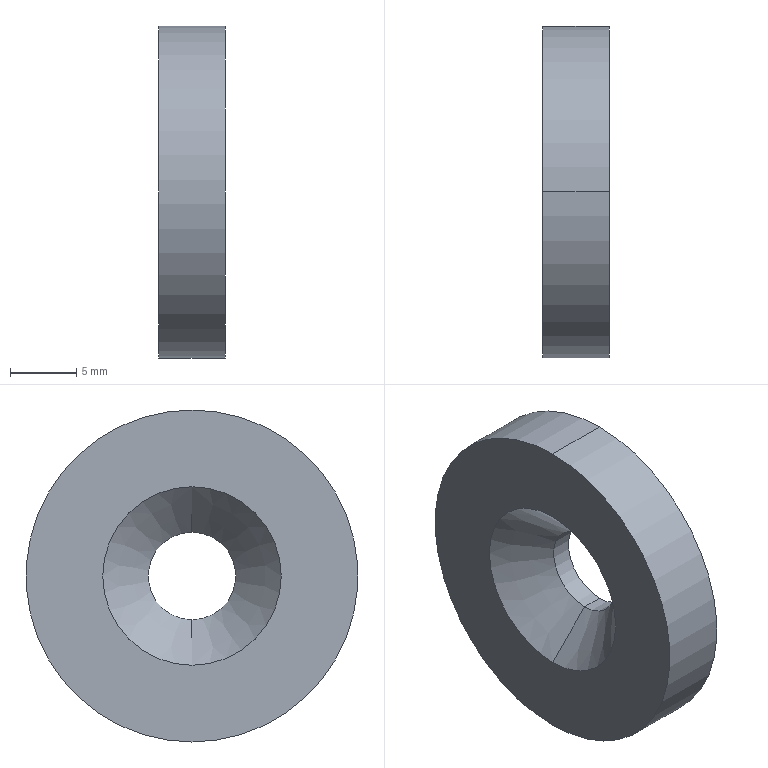Component | SolidWorks | EndCap1-1 | 1 solid | 8 faces | box 5 x 25 x 25 mm | volume 2120 mm3 | cylinder 4 | cone 2 | plane 2 | commonest cylinder face diameters 6.6 x2 25 x2
build123d program:
from build123d import *

# Parameters (mm, degrees)
SKETCH1_R                                            = 12.5
BOSS_EXTRUDE1_DEPTH                                  = 5
COUNTERSUNK_HOLE_FOR_M6_HEXAGON_SOCKET_C_D           = 6.6
COUNTERSUNK_HOLE_FOR_M6_HEXAGON_SOCKET_C_DEPTH       = 15
COUNTERSUNK_HOLE_FOR_M6_HEXAGON_SOCKET_C_CSINK_D     = 13.44
COUNTERSUNK_HOLE_FOR_M6_HEXAGON_SOCKET_C_CSINK_ANGLE = 90
COUNTERSUNK_HOLE_FOR_M6_HEXAGON_SOCKET_C_TIP         = 1.983


with BuildPart() as part:
    # Sketch1 → Boss-Extrude1 (new body)
    with BuildSketch(Plane.XY):
        Circle(SKETCH1_R)
    extrude(amount=BOSS_EXTRUDE1_DEPTH)

    # Countersunk Hole for M6 Hexagon Socket C
    with Locations(Plane.XY.offset(5)):
        with Locations((0, 0)):
            CounterSinkHole(COUNTERSUNK_HOLE_FOR_M6_HEXAGON_SOCKET_C_D / 2, COUNTERSUNK_HOLE_FOR_M6_HEXAGON_SOCKET_C_CSINK_D / 2, depth=COUNTERSUNK_HOLE_FOR_M6_HEXAGON_SOCKET_C_DEPTH, counter_sink_angle=COUNTERSUNK_HOLE_FOR_M6_HEXAGON_SOCKET_C_CSINK_ANGLE)
            with Locations((0, 0, -(COUNTERSUNK_HOLE_FOR_M6_HEXAGON_SOCKET_C_DEPTH + COUNTERSUNK_HOLE_FOR_M6_HEXAGON_SOCKET_C_TIP / 2))):  # 118° drill point
                Cone(0, COUNTERSUNK_HOLE_FOR_M6_HEXAGON_SOCKET_C_D / 2, COUNTERSUNK_HOLE_FOR_M6_HEXAGON_SOCKET_C_TIP, mode=Mode.SUBTRACT)


solid = part.part

# Placed as in the assembly
solid = solid.moved(Location((181.468, -65.334, 2056.399), (0, -90, 0)))
STEP:
#1=CARTESIAN_POINT('',(7.082,-2.572,80.831));
#2=VERTEX_POINT('',#1);
#3=CARTESIAN_POINT('',(7.082,-2.572,81.091));
#4=VERTEX_POINT('',#3);
#5=CARTESIAN_POINT('',(7.082,-2.572,80.961));
#6=DIRECTION('',(-1.,0.,-0.));
#7=DIRECTION('',(0.,0.,1.));
#8=AXIS2_PLACEMENT_3D('',#5,#6,#7);
#9=CIRCLE('',#8,0.1299);
#10=EDGE_CURVE('',#2,#4,#9,.T.);
#11=ORIENTED_EDGE('',*,*,#10,.F.);
#12=CARTESIAN_POINT('',(6.948,-2.572,80.696));
#13=VERTEX_POINT('',#12);
#14=CARTESIAN_POINT('',(6.948,-2.572,80.696));
#15=DIRECTION('',(-0.7071,0.,-0.7071));
#16=VECTOR('',#15,39.37);
#17=LINE('',#14,#16);
#18=EDGE_CURVE('',#2,#13,#17,.T.);
#19=ORIENTED_EDGE('',*,*,#18,.T.);
#20=CARTESIAN_POINT('',(6.948,-2.572,81.225));
#21=VERTEX_POINT('',#20);
#22=CARTESIAN_POINT('',(6.948,-2.572,80.961));
#23=DIRECTION('',(-1.,0.,-0.));
#24=DIRECTION('',(0.,0.,1.));
#25=AXIS2_PLACEMENT_3D('',#22,#23,#24);
#26=CIRCLE('',#25,0.2646);
#27=EDGE_CURVE('',#13,#21,#26,.T.);
#28=ORIENTED_EDGE('',*,*,#27,.T.);
#29=CARTESIAN_POINT('',(6.948,-2.572,81.225));
#30=DIRECTION('',(-0.7071,0.,0.7071));
#31=VECTOR('',#30,39.37);
#32=LINE('',#29,#31);
#33=EDGE_CURVE('',#4,#21,#32,.T.);
#34=ORIENTED_EDGE('',*,*,#33,.F.);
#35=EDGE_LOOP('',(#11,#19,#28,#34));
#36=FACE_OUTER_BOUND('',#35,.T.);
#37=CARTESIAN_POINT('',(6.948,-2.572,80.961));
#38=DIRECTION('',(-1.,0.,-0.));
#39=DIRECTION('',(0.,0.,1.));
#40=AXIS2_PLACEMENT_3D('',#37,#38,#39);
#41=CONICAL_SURFACE('',#40,0.2646,0.7854);
#42=ADVANCED_FACE('',(#36),#41,.F.);
#43=CARTESIAN_POINT('',(7.144,-2.572,80.831));
#44=VERTEX_POINT('',#43);
#45=CARTESIAN_POINT('',(7.144,-2.572,81.091));
#46=VERTEX_POINT('',#45);
#47=CARTESIAN_POINT('',(7.144,-2.572,80.961));
#48=DIRECTION('',(-1.,0.,-0.));
#49=DIRECTION('',(0.,0.,1.));
#50=AXIS2_PLACEMENT_3D('',#47,#48,#49);
#51=CIRCLE('',#50,0.1299);
#52=EDGE_CURVE('',#44,#46,#51,.T.);
#53=ORIENTED_EDGE('',*,*,#52,.F.);
#54=CARTESIAN_POINT('',(6.948,-2.572,80.831));
#55=DIRECTION('',(-1.,0.,-0.));
#56=VECTOR('',#55,39.37);
#57=LINE('',#54,#56);
#58=EDGE_CURVE('',#44,#2,#57,.T.);
#59=ORIENTED_EDGE('',*,*,#58,.T.);
#60=ORIENTED_EDGE('',*,*,#10,.T.);
#61=CARTESIAN_POINT('',(6.948,-2.572,81.091));
#62=DIRECTION('',(-1.,0.,-0.));
#63=VECTOR('',#62,39.37);
#64=LINE('',#61,#63);
#65=EDGE_CURVE('',#46,#4,#64,.T.);
#66=ORIENTED_EDGE('',*,*,#65,.F.);
#67=EDGE_LOOP('',(#53,#59,#60,#66));
#68=FACE_OUTER_BOUND('',#67,.T.);
#69=CARTESIAN_POINT('',(6.948,-2.572,80.961));
#70=DIRECTION('',(-1.,0.,-0.));
#71=DIRECTION('',(0.,0.,1.));
#72=AXIS2_PLACEMENT_3D('',#69,#70,#71);
#73=CYLINDRICAL_SURFACE('',#72,0.1299);
#74=ADVANCED_FACE('',(#68),#73,.F.);
#75=CARTESIAN_POINT('',(6.948,-2.572,81.453));
#76=VERTEX_POINT('',#75);
#77=CARTESIAN_POINT('',(6.948,-2.572,80.468));
#78=VERTEX_POINT('',#77);
#79=CARTESIAN_POINT('',(6.948,-2.572,80.961));
#80=DIRECTION('',(-1.,0.,-0.));
#81=DIRECTION('',(0.,0.,1.));
#82=AXIS2_PLACEMENT_3D('',#79,#80,#81);
#83=CIRCLE('',#82,0.4921);
#84=EDGE_CURVE('',#76,#78,#83,.T.);
#85=ORIENTED_EDGE('',*,*,#84,.F.);
#86=CARTESIAN_POINT('',(7.144,-2.572,81.453));
#87=VERTEX_POINT('',#86);
#88=CARTESIAN_POINT('',(6.948,-2.572,81.453));
#89=DIRECTION('',(1.,-0.,0.));
#90=VECTOR('',#89,39.37);
#91=LINE('',#88,#90);
#92=EDGE_CURVE('',#76,#87,#91,.T.);
#93=ORIENTED_EDGE('',*,*,#92,.T.);
#94=CARTESIAN_POINT('',(7.144,-2.572,80.468));
#95=VERTEX_POINT('',#94);
#96=CARTESIAN_POINT('',(7.144,-2.572,80.961));
#97=DIRECTION('',(-1.,0.,-0.));
#98=DIRECTION('',(0.,0.,1.));
#99=AXIS2_PLACEMENT_3D('',#96,#97,#98);
#100=CIRCLE('',#99,0.4921);
#101=EDGE_CURVE('',#87,#95,#100,.T.);
#102=ORIENTED_EDGE('',*,*,#101,.T.);
#103=CARTESIAN_POINT('',(6.948,-2.572,80.468));
#104=DIRECTION('',(1.,-0.,0.));
#105=VECTOR('',#104,39.37);
#106=LINE('',#103,#105);
#107=EDGE_CURVE('',#78,#95,#106,.T.);
#108=ORIENTED_EDGE('',*,*,#107,.F.);
#109=EDGE_LOOP('',(#85,#93,#102,#108));
#110=FACE_OUTER_BOUND('',#109,.T.);
#111=CARTESIAN_POINT('',(6.948,-2.572,80.961));
#112=DIRECTION('',(1.,-0.,0.));
#113=DIRECTION('',(0.,0.,-1.));
#114=AXIS2_PLACEMENT_3D('',#111,#112,#113);
#115=CYLINDRICAL_SURFACE('',#114,0.4921);
#116=ADVANCED_FACE('',(#110),#115,.T.);
#117=ORIENTED_EDGE('',*,*,#92,.F.);
#118=CARTESIAN_POINT('',(6.948,-2.572,80.961));
#119=DIRECTION('',(-1.,0.,-0.));
#120=DIRECTION('',(0.,0.,1.));
#121=AXIS2_PLACEMENT_3D('',#118,#119,#120);
#122=CIRCLE('',#121,0.4921);
#123=EDGE_CURVE('',#78,#76,#122,.T.);
#124=ORIENTED_EDGE('',*,*,#123,.F.);
#125=ORIENTED_EDGE('',*,*,#107,.T.);
#126=CARTESIAN_POINT('',(7.144,-2.572,80.961));
#127=DIRECTION('',(-1.,0.,-0.));
#128=DIRECTION('',(0.,0.,1.));
#129=AXIS2_PLACEMENT_3D('',#126,#127,#128);
#130=CIRCLE('',#129,0.4921);
#131=EDGE_CURVE('',#95,#87,#130,.T.);
#132=ORIENTED_EDGE('',*,*,#131,.T.);
#133=EDGE_LOOP('',(#117,#124,#125,#132));
#134=FACE_OUTER_BOUND('',#133,.T.);
#135=CARTESIAN_POINT('',(6.948,-2.572,80.961));
#136=DIRECTION('',(1.,-0.,0.));
#137=DIRECTION('',(0.,0.,-1.));
#138=AXIS2_PLACEMENT_3D('',#135,#136,#137);
#139=CYLINDRICAL_SURFACE('',#138,0.4921);
#140=ADVANCED_FACE('',(#134),#139,.T.);
#141=CARTESIAN_POINT('',(6.948,-2.572,80.961));
#142=DIRECTION('',(-1.,0.,-0.));
#143=DIRECTION('',(0.,0.,1.));
#144=AXIS2_PLACEMENT_3D('',#141,#142,#143);
#145=CIRCLE('',#144,0.2646);
#146=EDGE_CURVE('',#21,#13,#145,.T.);
#147=ORIENTED_EDGE('',*,*,#146,.F.);
#148=ORIENTED_EDGE('',*,*,#27,.F.);
#149=EDGE_LOOP('',(#147,#148));
#150=FACE_BOUND('',#149,.T.);
#151=ORIENTED_EDGE('',*,*,#123,.T.);
#152=ORIENTED_EDGE('',*,*,#84,.T.);
#153=EDGE_LOOP('',(#151,#152));
#154=FACE_OUTER_BOUND('',#153,.T.);
#155=CARTESIAN_POINT('',(6.948,-2.572,80.961));
#156=DIRECTION('',(-1.,0.,-0.));
#157=DIRECTION('',(-0.,0.,1.));
#158=AXIS2_PLACEMENT_3D('',#155,#156,#157);
#159=PLANE('',#158);
#160=ADVANCED_FACE('',(#150,#154),#159,.T.);
#161=CARTESIAN_POINT('',(7.144,-2.572,80.961));
#162=DIRECTION('',(-1.,0.,-0.));
#163=DIRECTION('',(0.,0.,1.));
#164=AXIS2_PLACEMENT_3D('',#161,#162,#163);
#165=CIRCLE('',#164,0.1299);
#166=EDGE_CURVE('',#46,#44,#165,.T.);
#167=ORIENTED_EDGE('',*,*,#166,.T.);
#168=ORIENTED_EDGE('',*,*,#52,.T.);
#169=EDGE_LOOP('',(#167,#168));
#170=FACE_BOUND('',#169,.T.);
#171=ORIENTED_EDGE('',*,*,#131,.F.);
#172=ORIENTED_EDGE('',*,*,#101,.F.);
#173=EDGE_LOOP('',(#171,#172));
#174=FACE_OUTER_BOUND('',#173,.T.);
#175=CARTESIAN_POINT('',(7.144,-2.572,80.961));
#176=DIRECTION('',(-1.,0.,-0.));
#177=DIRECTION('',(-0.,0.,1.));
#178=AXIS2_PLACEMENT_3D('',#175,#176,#177);
#179=PLANE('',#178);
#180=ADVANCED_FACE('',(#170,#174),#179,.F.);
#181=ORIENTED_EDGE('',*,*,#58,.F.);
#182=ORIENTED_EDGE('',*,*,#166,.F.);
#183=ORIENTED_EDGE('',*,*,#65,.T.);
#184=CARTESIAN_POINT('',(7.082,-2.572,80.961));
#185=DIRECTION('',(-1.,0.,-0.));
#186=DIRECTION('',(0.,0.,1.));
#187=AXIS2_PLACEMENT_3D('',#184,#185,#186);
#188=CIRCLE('',#187,0.1299);
#189=EDGE_CURVE('',#4,#2,#188,.T.);
#190=ORIENTED_EDGE('',*,*,#189,.T.);
#191=EDGE_LOOP('',(#181,#182,#183,#190));
#192=FACE_OUTER_BOUND('',#191,.T.);
#193=CARTESIAN_POINT('',(6.948,-2.572,80.961));
#194=DIRECTION('',(-1.,0.,-0.));
#195=DIRECTION('',(0.,0.,1.));
#196=AXIS2_PLACEMENT_3D('',#193,#194,#195);
#197=CYLINDRICAL_SURFACE('',#196,0.1299);
#198=ADVANCED_FACE('',(#192),#197,.F.);
#199=ORIENTED_EDGE('',*,*,#18,.F.);
#200=ORIENTED_EDGE('',*,*,#189,.F.);
#201=ORIENTED_EDGE('',*,*,#33,.T.);
#202=ORIENTED_EDGE('',*,*,#146,.T.);
#203=EDGE_LOOP('',(#199,#200,#201,#202));
#204=FACE_OUTER_BOUND('',#203,.T.);
#205=CARTESIAN_POINT('',(6.948,-2.572,80.961));
#206=DIRECTION('',(-1.,0.,-0.));
#207=DIRECTION('',(0.,0.,1.));
#208=AXIS2_PLACEMENT_3D('',#205,#206,#207);
#209=CONICAL_SURFACE('',#208,0.2646,0.7854);
#210=ADVANCED_FACE('',(#204),#209,.F.);
#211=CLOSED_SHELL('',(#42,#74,#116,#140,#160,#180,#198,#210));
#212=MANIFOLD_SOLID_BREP('',#211);
#213=CARTESIAN_POINT('',(0.,0.,0.));
#214=DIRECTION('',(0.,0.,1.));
#215=DIRECTION('',(1.,0.,0.));
#216=AXIS2_PLACEMENT_3D('',#213,#214,#215);
#217=(LENGTH_UNIT()NAMED_UNIT(*)SI_UNIT($,.METRE.));
#218=LENGTH_MEASURE_WITH_UNIT(LENGTH_MEASURE(0.0254),#217);
#219=DIMENSIONAL_EXPONENTS(1.,0.,0.,0.,0.,0.,0.);
#220=(CONVERSION_BASED_UNIT('',#218)LENGTH_UNIT()NAMED_UNIT(#219));
#221=UNCERTAINTY_MEASURE_WITH_UNIT(LENGTH_MEASURE(0.00001),#220,'','');
#222=(NAMED_UNIT(*)PLANE_ANGLE_UNIT()SI_UNIT($,.RADIAN.));
#223=(NAMED_UNIT(*)SI_UNIT($,.STERADIAN.)SOLID_ANGLE_UNIT());
#224=(GEOMETRIC_REPRESENTATION_CONTEXT(3)GLOBAL_UNCERTAINTY_ASSIGNED_CONTEXT((#221))GLOBAL_UNIT_ASSIGNED_CONTEXT((#220,#222,#223))REPRESENTATION_CONTEXT('',''));
#225=ADVANCED_BREP_SHAPE_REPRESENTATION('',(#212,#216),#224);
#226=COLOUR_RGB('',0.7922,0.8196,0.9333);
#227=FILL_AREA_STYLE_COLOUR('',#226);
#228=FILL_AREA_STYLE('',(#227));
#229=SURFACE_STYLE_FILL_AREA(#228);
#230=SURFACE_SIDE_STYLE('',(#229));
#231=SURFACE_STYLE_USAGE(.BOTH.,#230);
#232=PRESENTATION_STYLE_ASSIGNMENT((#231));
#233=STYLED_ITEM('',(#232),#212);
#234=(LENGTH_UNIT()NAMED_UNIT(*)SI_UNIT($,.METRE.));
#235=LENGTH_MEASURE_WITH_UNIT(LENGTH_MEASURE(0.0254),#234);
#236=DIMENSIONAL_EXPONENTS(1.,0.,0.,0.,0.,0.,0.);
#237=(CONVERSION_BASED_UNIT('',#235)LENGTH_UNIT()NAMED_UNIT(#236));
#238=UNCERTAINTY_MEASURE_WITH_UNIT(LENGTH_MEASURE(0.00001),#237,'','');
#239=(NAMED_UNIT(*)PLANE_ANGLE_UNIT()SI_UNIT($,.RADIAN.));
#240=(NAMED_UNIT(*)SI_UNIT($,.STERADIAN.)SOLID_ANGLE_UNIT());
#241=(GEOMETRIC_REPRESENTATION_CONTEXT(3)GLOBAL_UNCERTAINTY_ASSIGNED_CONTEXT((#238))GLOBAL_UNIT_ASSIGNED_CONTEXT((#237,#239,#240))REPRESENTATION_CONTEXT('',''));
#242=MECHANICAL_DESIGN_GEOMETRIC_PRESENTATION_REPRESENTATION('',(#233),#241);
#243=PRESENTATION_LAYER_ASSIGNMENT('','',(#233));